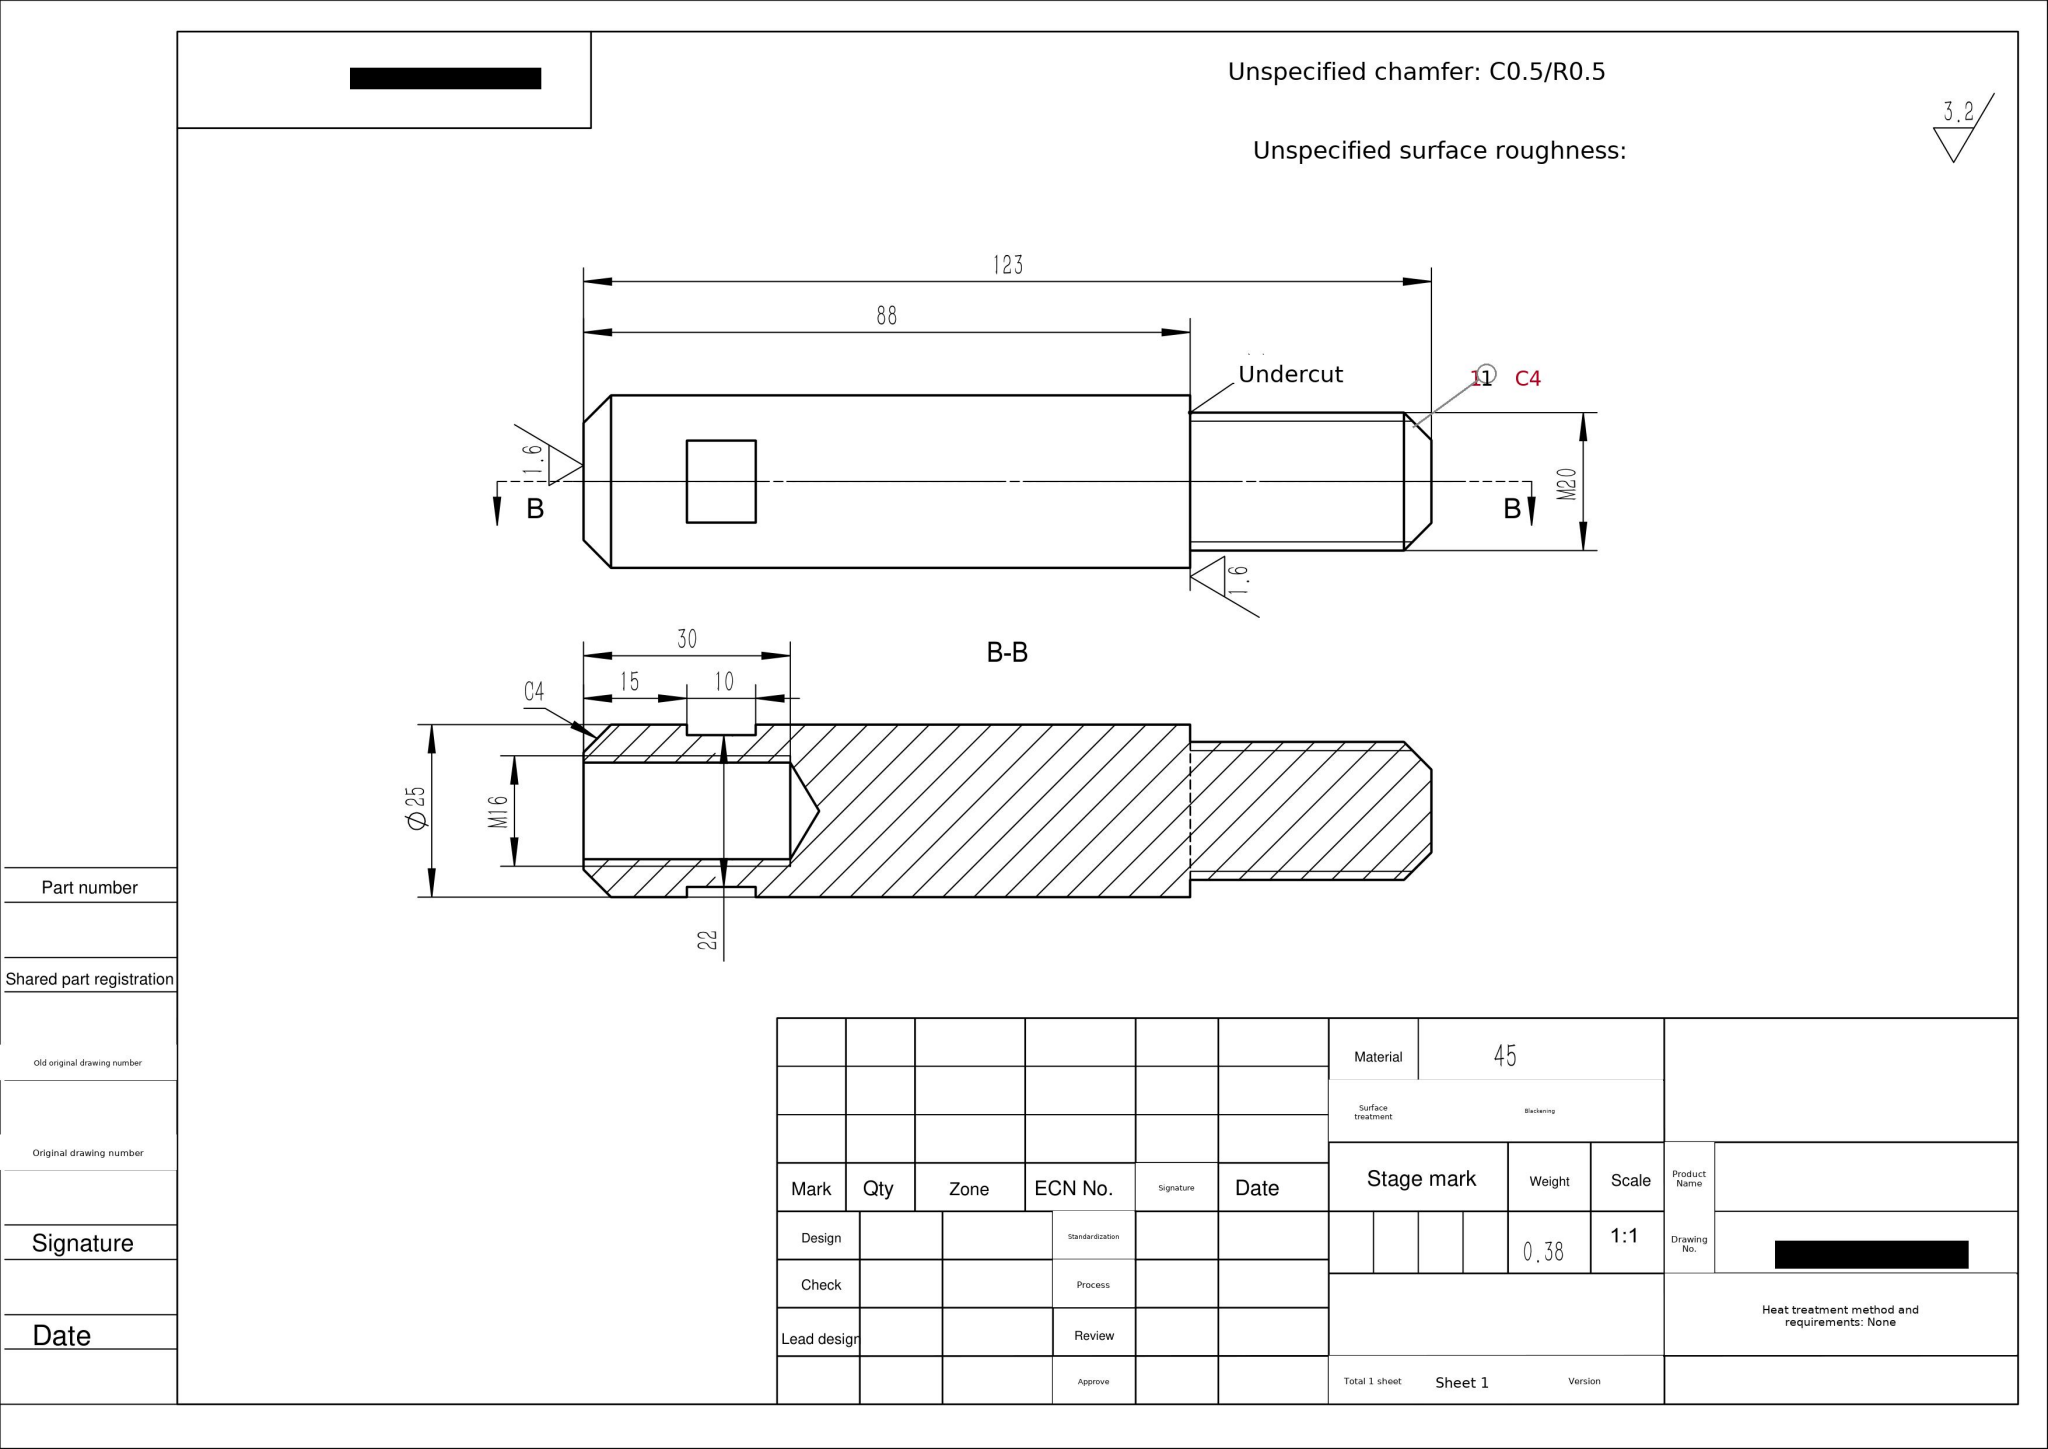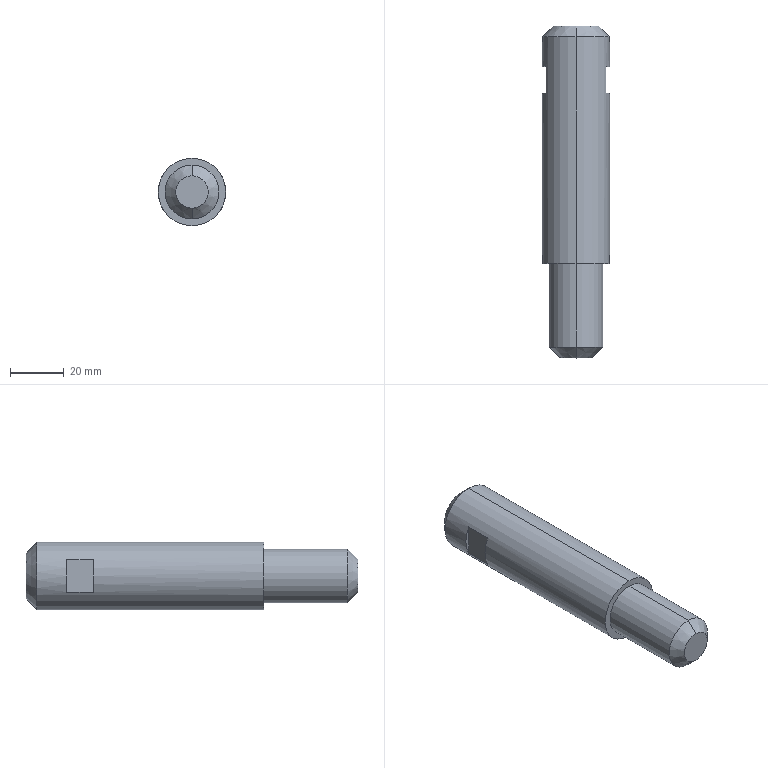Part | SolidWorks | mm | material 45 | 1 solid | 21 faces | box 25 x 123 x 25 mm | volume 48121 mm3 | plane 9 | cylinder 6 | cone 6 | commonest cylinder face diameters 14 x2 20 x2 25 x2
build123d program:
from build123d import *

# Parameters (mm, degrees)
SKETCH1_R              = 12.5
BOSS_EXTRUDE1_DEPTH    = 123
SKETCH2_OUTSIDE_W      = 52.596
SKETCH2_OUTSIDE_H      = 52.596
SKETCH2_OUTSIDE_R      = 10
CUT_EXTRUDE1_DEPTH     = 35
CHAMFER1_SIZE          = 4
M16_TAPPED_HOLE1_D     = 14
M16_TAPPED_HOLE1_DEPTH = 30
M16_TAPPED_HOLE1_TIP   = 4.206
CUT_EXTRUDE2_START     = -15
SKETCH8_OUTSIDE_W      = 52.596
SKETCH8_OUTSIDE_H      = 52.596
SKETCH8_OUTSIDE_W_2    = 22
SKETCH8_OUTSIDE_H_2    = 26.005
CUT_EXTRUDE2_DEPTH     = 10


with BuildPart() as part:
    # Sketch1 → Boss-Extrude1 (new body)
    with BuildSketch(Plane(origin=(0, 0, 0), x_dir=(1, 0, 0), z_dir=(0, 1, 0))):
        with Locations(Location((0, 0, 0), (0, 0, 270))):
            Circle(SKETCH1_R)
    extrude(amount=BOSS_EXTRUDE1_DEPTH)

    # Sketch2 outside → Cut-Extrude1 (cut)
    with BuildSketch(Plane.XZ):
        Rectangle(SKETCH2_OUTSIDE_W, SKETCH2_OUTSIDE_H)
        with Locations(Location((0, 0, 0), (0, 0, 270))):
            Circle(SKETCH2_OUTSIDE_R, mode=Mode.SUBTRACT)
    extrude(amount=-CUT_EXTRUDE1_DEPTH, mode=Mode.SUBTRACT)

    # Chamfer1
    chamfer1_edges = [part.edges().sort_by_distance(p)[0] for p in [
        (0, 0, 10),
        (0, 123, -12.5),
    ]]
    chamfer(chamfer1_edges, length=CHAMFER1_SIZE)

    # M16 Tapped Hole1
    with Locations(Plane(origin=(0, 123, 0), x_dir=(1, 0, 0), z_dir=(0, 1, 0))):
        with Locations((0, 0)):
            Hole(M16_TAPPED_HOLE1_D / 2, depth=M16_TAPPED_HOLE1_DEPTH)
            with Locations((0, 0, -(M16_TAPPED_HOLE1_DEPTH + M16_TAPPED_HOLE1_TIP / 2))):  # 118° drill point
                Cone(0, M16_TAPPED_HOLE1_D / 2, M16_TAPPED_HOLE1_TIP, mode=Mode.SUBTRACT)

    # Sketch8 outside → Cut-Extrude2 (cut)
    with BuildSketch(Plane(origin=(0, 123, 0), x_dir=(1, 0, 0), z_dir=(0, 1, 0)).offset(CUT_EXTRUDE2_START)):
        Rectangle(SKETCH8_OUTSIDE_W, SKETCH8_OUTSIDE_H)
        Rectangle(SKETCH8_OUTSIDE_W_2, SKETCH8_OUTSIDE_H_2, mode=Mode.SUBTRACT)
    extrude(amount=-CUT_EXTRUDE2_DEPTH, mode=Mode.SUBTRACT)


solid = part.part
STEP:
#1=CARTESIAN_POINT('',(0.,93.,-7.));
#2=VERTEX_POINT('',#1);
#3=CARTESIAN_POINT('',(0.,93.,7.));
#4=VERTEX_POINT('',#3);
#5=CARTESIAN_POINT('',(0.,93.,0.));
#6=DIRECTION('',(0.,1.,0.));
#7=DIRECTION('',(0.,0.,1.));
#8=AXIS2_PLACEMENT_3D('',#5,#6,#7);
#9=CIRCLE('',#8,7.);
#10=EDGE_CURVE('',#2,#4,#9,.T.);
#11=ORIENTED_EDGE('',*,*,#10,.F.);
#12=CARTESIAN_POINT('',(0.,123.,-7.));
#13=VERTEX_POINT('',#12);
#14=CARTESIAN_POINT('',(0.,123.,-7.));
#15=DIRECTION('',(0.,1.,0.));
#16=VECTOR('',#15,1000.);
#17=LINE('',#14,#16);
#18=EDGE_CURVE('',#2,#13,#17,.T.);
#19=ORIENTED_EDGE('',*,*,#18,.T.);
#20=CARTESIAN_POINT('',(0.,123.,7.));
#21=VERTEX_POINT('',#20);
#22=CARTESIAN_POINT('',(0.,123.,0.));
#23=DIRECTION('',(0.,1.,0.));
#24=DIRECTION('',(0.,0.,1.));
#25=AXIS2_PLACEMENT_3D('',#22,#23,#24);
#26=CIRCLE('',#25,7.);
#27=EDGE_CURVE('',#13,#21,#26,.T.);
#28=ORIENTED_EDGE('',*,*,#27,.T.);
#29=CARTESIAN_POINT('',(0.,123.,7.));
#30=DIRECTION('',(0.,1.,0.));
#31=VECTOR('',#30,1000.);
#32=LINE('',#29,#31);
#33=EDGE_CURVE('',#4,#21,#32,.T.);
#34=ORIENTED_EDGE('',*,*,#33,.F.);
#35=EDGE_LOOP('',(#11,#19,#28,#34));
#36=FACE_OUTER_BOUND('',#35,.T.);
#37=CARTESIAN_POINT('',(0.,123.,0.));
#38=DIRECTION('',(0.,1.,0.));
#39=DIRECTION('',(0.,0.,1.));
#40=AXIS2_PLACEMENT_3D('',#37,#38,#39);
#41=CYLINDRICAL_SURFACE('',#40,7.);
#42=ADVANCED_FACE('',(#36),#41,.F.);
#43=CARTESIAN_POINT('',(-0.,88.794,0.));
#44=VERTEX_POINT('',#43);
#45=CARTESIAN_POINT('',(0.,93.,7.));
#46=DIRECTION('',(0.,0.515,0.8572));
#47=VECTOR('',#46,1000.);
#48=LINE('',#45,#47);
#49=EDGE_CURVE('',#44,#4,#48,.T.);
#50=ORIENTED_EDGE('',*,*,#49,.F.);
#51=CARTESIAN_POINT('',(0.,93.,-7.));
#52=DIRECTION('',(0.,0.515,-0.8572));
#53=VECTOR('',#52,1000.);
#54=LINE('',#51,#53);
#55=EDGE_CURVE('',#44,#2,#54,.T.);
#56=ORIENTED_EDGE('',*,*,#55,.T.);
#57=ORIENTED_EDGE('',*,*,#10,.T.);
#58=EDGE_LOOP('',(#50,#56,#57));
#59=FACE_OUTER_BOUND('',#58,.T.);
#60=CARTESIAN_POINT('',(0.,93.,0.));
#61=DIRECTION('',(0.,1.,0.));
#62=DIRECTION('',(0.,0.,1.));
#63=AXIS2_PLACEMENT_3D('',#60,#61,#62);
#64=CONICAL_SURFACE('',#63,7.,1.03);
#65=ADVANCED_FACE('',(#59),#64,.F.);
#66=CARTESIAN_POINT('',(0.,0.,-6.));
#67=VERTEX_POINT('',#66);
#68=CARTESIAN_POINT('',(0.,0.,6.));
#69=VERTEX_POINT('',#68);
#70=CARTESIAN_POINT('',(0.,0.,0.));
#71=DIRECTION('',(0.,-1.,0.));
#72=DIRECTION('',(0.,0.,1.));
#73=AXIS2_PLACEMENT_3D('',#70,#71,#72);
#74=CIRCLE('',#73,6.);
#75=EDGE_CURVE('',#67,#69,#74,.T.);
#76=ORIENTED_EDGE('',*,*,#75,.F.);
#77=CARTESIAN_POINT('',(0.,4.,-10.));
#78=VERTEX_POINT('',#77);
#79=CARTESIAN_POINT('',(0.,0.,-6.));
#80=DIRECTION('',(0.,0.7071,-0.7071));
#81=VECTOR('',#80,1000.);
#82=LINE('',#79,#81);
#83=EDGE_CURVE('',#67,#78,#82,.T.);
#84=ORIENTED_EDGE('',*,*,#83,.T.);
#85=CARTESIAN_POINT('',(0.,4.,10.));
#86=VERTEX_POINT('',#85);
#87=CARTESIAN_POINT('',(0.,4.,0.));
#88=DIRECTION('',(0.,1.,0.));
#89=DIRECTION('',(0.,0.,1.));
#90=AXIS2_PLACEMENT_3D('',#87,#88,#89);
#91=CIRCLE('',#90,10.);
#92=EDGE_CURVE('',#86,#78,#91,.T.);
#93=ORIENTED_EDGE('',*,*,#92,.F.);
#94=CARTESIAN_POINT('',(0.,0.,6.));
#95=DIRECTION('',(0.,0.7071,0.7071));
#96=VECTOR('',#95,1000.);
#97=LINE('',#94,#96);
#98=EDGE_CURVE('',#69,#86,#97,.T.);
#99=ORIENTED_EDGE('',*,*,#98,.F.);
#100=EDGE_LOOP('',(#76,#84,#93,#99));
#101=FACE_OUTER_BOUND('',#100,.T.);
#102=CARTESIAN_POINT('',(0.,0.,0.));
#103=DIRECTION('',(0.,1.,0.));
#104=DIRECTION('',(0.,0.,1.));
#105=AXIS2_PLACEMENT_3D('',#102,#103,#104);
#106=CONICAL_SURFACE('',#105,6.,0.7854);
#107=ADVANCED_FACE('',(#101),#106,.T.);
#108=CARTESIAN_POINT('',(0.,123.,8.5));
#109=VERTEX_POINT('',#108);
#110=CARTESIAN_POINT('',(0.,123.,-8.5));
#111=VERTEX_POINT('',#110);
#112=CARTESIAN_POINT('',(0.,123.,0.));
#113=DIRECTION('',(0.,1.,0.));
#114=DIRECTION('',(0.,0.,1.));
#115=AXIS2_PLACEMENT_3D('',#112,#113,#114);
#116=CIRCLE('',#115,8.5);
#117=EDGE_CURVE('',#109,#111,#116,.T.);
#118=ORIENTED_EDGE('',*,*,#117,.F.);
#119=CARTESIAN_POINT('',(0.,119.,12.5));
#120=VERTEX_POINT('',#119);
#121=CARTESIAN_POINT('',(0.,123.,8.5));
#122=DIRECTION('',(0.,-0.7071,0.7071));
#123=VECTOR('',#122,1000.);
#124=LINE('',#121,#123);
#125=EDGE_CURVE('',#109,#120,#124,.T.);
#126=ORIENTED_EDGE('',*,*,#125,.T.);
#127=CARTESIAN_POINT('',(0.,119.,-12.5));
#128=VERTEX_POINT('',#127);
#129=CARTESIAN_POINT('',(0.,119.,0.));
#130=DIRECTION('',(0.,-1.,0.));
#131=DIRECTION('',(0.,0.,1.));
#132=AXIS2_PLACEMENT_3D('',#129,#130,#131);
#133=CIRCLE('',#132,12.5);
#134=EDGE_CURVE('',#128,#120,#133,.T.);
#135=ORIENTED_EDGE('',*,*,#134,.F.);
#136=CARTESIAN_POINT('',(0.,123.,-8.5));
#137=DIRECTION('',(0.,-0.7071,-0.7071));
#138=VECTOR('',#137,1000.);
#139=LINE('',#136,#138);
#140=EDGE_CURVE('',#111,#128,#139,.T.);
#141=ORIENTED_EDGE('',*,*,#140,.F.);
#142=EDGE_LOOP('',(#118,#126,#135,#141));
#143=FACE_OUTER_BOUND('',#142,.T.);
#144=CARTESIAN_POINT('',(0.,123.,0.));
#145=DIRECTION('',(0.,-1.,0.));
#146=DIRECTION('',(0.,0.,-1.));
#147=AXIS2_PLACEMENT_3D('',#144,#145,#146);
#148=CONICAL_SURFACE('',#147,8.5,0.7854);
#149=ADVANCED_FACE('',(#143),#148,.T.);
#150=CARTESIAN_POINT('',(0.,35.,-10.));
#151=VERTEX_POINT('',#150);
#152=CARTESIAN_POINT('',(0.,35.,10.));
#153=VERTEX_POINT('',#152);
#154=CARTESIAN_POINT('',(0.,35.,0.));
#155=DIRECTION('',(0.,-1.,0.));
#156=DIRECTION('',(0.,0.,-1.));
#157=AXIS2_PLACEMENT_3D('',#154,#155,#156);
#158=CIRCLE('',#157,10.);
#159=EDGE_CURVE('',#151,#153,#158,.T.);
#160=ORIENTED_EDGE('',*,*,#159,.T.);
#161=CARTESIAN_POINT('',(0.,35.,10.));
#162=DIRECTION('',(0.,-1.,0.));
#163=VECTOR('',#162,1000.);
#164=LINE('',#161,#163);
#165=EDGE_CURVE('',#153,#86,#164,.T.);
#166=ORIENTED_EDGE('',*,*,#165,.T.);
#167=ORIENTED_EDGE('',*,*,#92,.T.);
#168=CARTESIAN_POINT('',(0.,35.,-10.));
#169=DIRECTION('',(0.,-1.,0.));
#170=VECTOR('',#169,1000.);
#171=LINE('',#168,#170);
#172=EDGE_CURVE('',#151,#78,#171,.T.);
#173=ORIENTED_EDGE('',*,*,#172,.F.);
#174=EDGE_LOOP('',(#160,#166,#167,#173));
#175=FACE_OUTER_BOUND('',#174,.T.);
#176=CARTESIAN_POINT('',(0.,35.,0.));
#177=DIRECTION('',(0.,-1.,0.));
#178=DIRECTION('',(0.,0.,-1.));
#179=AXIS2_PLACEMENT_3D('',#176,#177,#178);
#180=CYLINDRICAL_SURFACE('',#179,10.);
#181=ADVANCED_FACE('',(#175),#180,.T.);
#182=CARTESIAN_POINT('',(11.,108.,5.937));
#183=VERTEX_POINT('',#182);
#184=CARTESIAN_POINT('',(11.,98.,5.937));
#185=VERTEX_POINT('',#184);
#186=CARTESIAN_POINT('',(11.,123.,5.937));
#187=DIRECTION('',(0.,-1.,0.));
#188=VECTOR('',#187,1000.);
#189=LINE('',#186,#188);
#190=EDGE_CURVE('',#183,#185,#189,.T.);
#191=ORIENTED_EDGE('',*,*,#190,.F.);
#192=CARTESIAN_POINT('',(11.,108.,-5.937));
#193=VERTEX_POINT('',#192);
#194=CARTESIAN_POINT('',(0.,108.,0.));
#195=DIRECTION('',(0.,1.,0.));
#196=DIRECTION('',(0.,0.,1.));
#197=AXIS2_PLACEMENT_3D('',#194,#195,#196);
#198=CIRCLE('',#197,12.5);
#199=EDGE_CURVE('',#183,#193,#198,.T.);
#200=ORIENTED_EDGE('',*,*,#199,.T.);
#201=CARTESIAN_POINT('',(11.,98.,-5.937));
#202=VERTEX_POINT('',#201);
#203=CARTESIAN_POINT('',(11.,123.,-5.937));
#204=DIRECTION('',(0.,1.,0.));
#205=VECTOR('',#204,1000.);
#206=LINE('',#203,#205);
#207=EDGE_CURVE('',#202,#193,#206,.T.);
#208=ORIENTED_EDGE('',*,*,#207,.F.);
#209=CARTESIAN_POINT('',(0.,98.,0.));
#210=DIRECTION('',(0.,1.,0.));
#211=DIRECTION('',(0.,0.,1.));
#212=AXIS2_PLACEMENT_3D('',#209,#210,#211);
#213=CIRCLE('',#212,12.5);
#214=EDGE_CURVE('',#185,#202,#213,.T.);
#215=ORIENTED_EDGE('',*,*,#214,.F.);
#216=EDGE_LOOP('',(#191,#200,#208,#215));
#217=FACE_BOUND('',#216,.T.);
#218=ORIENTED_EDGE('',*,*,#134,.T.);
#219=CARTESIAN_POINT('',(0.,35.,12.5));
#220=VERTEX_POINT('',#219);
#221=CARTESIAN_POINT('',(0.,123.,12.5));
#222=DIRECTION('',(0.,-1.,0.));
#223=VECTOR('',#222,1000.);
#224=LINE('',#221,#223);
#225=EDGE_CURVE('',#120,#220,#224,.T.);
#226=ORIENTED_EDGE('',*,*,#225,.T.);
#227=CARTESIAN_POINT('',(0.,35.,-12.5));
#228=VERTEX_POINT('',#227);
#229=CARTESIAN_POINT('',(0.,35.,0.));
#230=DIRECTION('',(0.,-1.,0.));
#231=DIRECTION('',(0.,0.,-1.));
#232=AXIS2_PLACEMENT_3D('',#229,#230,#231);
#233=CIRCLE('',#232,12.5);
#234=EDGE_CURVE('',#228,#220,#233,.T.);
#235=ORIENTED_EDGE('',*,*,#234,.F.);
#236=CARTESIAN_POINT('',(0.,123.,-12.5));
#237=DIRECTION('',(0.,-1.,0.));
#238=VECTOR('',#237,1000.);
#239=LINE('',#236,#238);
#240=EDGE_CURVE('',#128,#228,#239,.T.);
#241=ORIENTED_EDGE('',*,*,#240,.F.);
#242=EDGE_LOOP('',(#218,#226,#235,#241));
#243=FACE_OUTER_BOUND('',#242,.T.);
#244=CARTESIAN_POINT('',(0.,123.,0.));
#245=DIRECTION('',(0.,-1.,0.));
#246=DIRECTION('',(0.,0.,-1.));
#247=AXIS2_PLACEMENT_3D('',#244,#245,#246);
#248=CYLINDRICAL_SURFACE('',#247,12.5);
#249=ADVANCED_FACE('',(#217,#243),#248,.T.);
#250=ORIENTED_EDGE('',*,*,#225,.F.);
#251=CARTESIAN_POINT('',(0.,119.,0.));
#252=DIRECTION('',(0.,-1.,0.));
#253=DIRECTION('',(0.,0.,1.));
#254=AXIS2_PLACEMENT_3D('',#251,#252,#253);
#255=CIRCLE('',#254,12.5);
#256=EDGE_CURVE('',#120,#128,#255,.T.);
#257=ORIENTED_EDGE('',*,*,#256,.T.);
#258=ORIENTED_EDGE('',*,*,#240,.T.);
#259=CARTESIAN_POINT('',(0.,35.,0.));
#260=DIRECTION('',(0.,-1.,0.));
#261=DIRECTION('',(0.,0.,-1.));
#262=AXIS2_PLACEMENT_3D('',#259,#260,#261);
#263=CIRCLE('',#262,12.5);
#264=EDGE_CURVE('',#220,#228,#263,.T.);
#265=ORIENTED_EDGE('',*,*,#264,.F.);
#266=EDGE_LOOP('',(#250,#257,#258,#265));
#267=FACE_OUTER_BOUND('',#266,.T.);
#268=CARTESIAN_POINT('',(-11.,108.,-5.937));
#269=VERTEX_POINT('',#268);
#270=CARTESIAN_POINT('',(-11.,98.,-5.937));
#271=VERTEX_POINT('',#270);
#272=CARTESIAN_POINT('',(-11.,123.,-5.937));
#273=DIRECTION('',(0.,-1.,0.));
#274=VECTOR('',#273,1000.);
#275=LINE('',#272,#274);
#276=EDGE_CURVE('',#269,#271,#275,.T.);
#277=ORIENTED_EDGE('',*,*,#276,.F.);
#278=CARTESIAN_POINT('',(-11.,108.,5.937));
#279=VERTEX_POINT('',#278);
#280=CARTESIAN_POINT('',(0.,108.,0.));
#281=DIRECTION('',(0.,1.,0.));
#282=DIRECTION('',(0.,0.,1.));
#283=AXIS2_PLACEMENT_3D('',#280,#281,#282);
#284=CIRCLE('',#283,12.5);
#285=EDGE_CURVE('',#269,#279,#284,.T.);
#286=ORIENTED_EDGE('',*,*,#285,.T.);
#287=CARTESIAN_POINT('',(-11.,98.,5.937));
#288=VERTEX_POINT('',#287);
#289=CARTESIAN_POINT('',(-11.,123.,5.937));
#290=DIRECTION('',(0.,1.,0.));
#291=VECTOR('',#290,1000.);
#292=LINE('',#289,#291);
#293=EDGE_CURVE('',#288,#279,#292,.T.);
#294=ORIENTED_EDGE('',*,*,#293,.F.);
#295=CARTESIAN_POINT('',(0.,98.,0.));
#296=DIRECTION('',(0.,1.,0.));
#297=DIRECTION('',(0.,0.,1.));
#298=AXIS2_PLACEMENT_3D('',#295,#296,#297);
#299=CIRCLE('',#298,12.5);
#300=EDGE_CURVE('',#271,#288,#299,.T.);
#301=ORIENTED_EDGE('',*,*,#300,.F.);
#302=EDGE_LOOP('',(#277,#286,#294,#301));
#303=FACE_BOUND('',#302,.T.);
#304=CARTESIAN_POINT('',(0.,123.,0.));
#305=DIRECTION('',(0.,-1.,0.));
#306=DIRECTION('',(0.,0.,-1.));
#307=AXIS2_PLACEMENT_3D('',#304,#305,#306);
#308=CYLINDRICAL_SURFACE('',#307,12.5);
#309=ADVANCED_FACE('',(#267,#303),#308,.T.);
#310=CARTESIAN_POINT('',(0.,123.,0.));
#311=DIRECTION('',(0.,1.,0.));
#312=DIRECTION('',(0.,0.,1.));
#313=AXIS2_PLACEMENT_3D('',#310,#311,#312);
#314=CIRCLE('',#313,7.);
#315=EDGE_CURVE('',#21,#13,#314,.T.);
#316=ORIENTED_EDGE('',*,*,#315,.F.);
#317=ORIENTED_EDGE('',*,*,#27,.F.);
#318=EDGE_LOOP('',(#316,#317));
#319=FACE_BOUND('',#318,.T.);
#320=CARTESIAN_POINT('',(0.,123.,0.));
#321=DIRECTION('',(0.,1.,0.));
#322=DIRECTION('',(0.,0.,1.));
#323=AXIS2_PLACEMENT_3D('',#320,#321,#322);
#324=CIRCLE('',#323,8.5);
#325=EDGE_CURVE('',#111,#109,#324,.T.);
#326=ORIENTED_EDGE('',*,*,#325,.T.);
#327=ORIENTED_EDGE('',*,*,#117,.T.);
#328=EDGE_LOOP('',(#326,#327));
#329=FACE_OUTER_BOUND('',#328,.T.);
#330=CARTESIAN_POINT('',(0.,123.,0.));
#331=DIRECTION('',(0.,1.,0.));
#332=DIRECTION('',(0.,0.,1.));
#333=AXIS2_PLACEMENT_3D('',#330,#331,#332);
#334=PLANE('',#333);
#335=ADVANCED_FACE('',(#319,#329),#334,.T.);
#336=ORIENTED_EDGE('',*,*,#159,.F.);
#337=CARTESIAN_POINT('',(0.,35.,0.));
#338=DIRECTION('',(0.,-1.,0.));
#339=DIRECTION('',(0.,0.,-1.));
#340=AXIS2_PLACEMENT_3D('',#337,#338,#339);
#341=CIRCLE('',#340,10.);
#342=EDGE_CURVE('',#153,#151,#341,.T.);
#343=ORIENTED_EDGE('',*,*,#342,.F.);
#344=EDGE_LOOP('',(#336,#343));
#345=FACE_BOUND('',#344,.T.);
#346=ORIENTED_EDGE('',*,*,#234,.T.);
#347=ORIENTED_EDGE('',*,*,#264,.T.);
#348=EDGE_LOOP('',(#346,#347));
#349=FACE_OUTER_BOUND('',#348,.T.);
#350=CARTESIAN_POINT('',(0.,35.,0.));
#351=DIRECTION('',(0.,-1.,0.));
#352=DIRECTION('',(0.,0.,-1.));
#353=AXIS2_PLACEMENT_3D('',#350,#351,#352);
#354=PLANE('',#353);
#355=ADVANCED_FACE('',(#345,#349),#354,.T.);
#356=ORIENTED_EDGE('',*,*,#165,.F.);
#357=ORIENTED_EDGE('',*,*,#342,.T.);
#358=ORIENTED_EDGE('',*,*,#172,.T.);
#359=CARTESIAN_POINT('',(0.,4.,0.));
#360=DIRECTION('',(0.,1.,0.));
#361=DIRECTION('',(0.,0.,1.));
#362=AXIS2_PLACEMENT_3D('',#359,#360,#361);
#363=CIRCLE('',#362,10.);
#364=EDGE_CURVE('',#78,#86,#363,.T.);
#365=ORIENTED_EDGE('',*,*,#364,.T.);
#366=EDGE_LOOP('',(#356,#357,#358,#365));
#367=FACE_OUTER_BOUND('',#366,.T.);
#368=CARTESIAN_POINT('',(0.,35.,0.));
#369=DIRECTION('',(0.,-1.,0.));
#370=DIRECTION('',(0.,0.,-1.));
#371=AXIS2_PLACEMENT_3D('',#368,#369,#370);
#372=CYLINDRICAL_SURFACE('',#371,10.);
#373=ADVANCED_FACE('',(#367),#372,.T.);
#374=CARTESIAN_POINT('',(0.,0.,0.));
#375=DIRECTION('',(0.,-1.,0.));
#376=DIRECTION('',(0.,0.,1.));
#377=AXIS2_PLACEMENT_3D('',#374,#375,#376);
#378=CIRCLE('',#377,6.);
#379=EDGE_CURVE('',#69,#67,#378,.T.);
#380=ORIENTED_EDGE('',*,*,#379,.T.);
#381=ORIENTED_EDGE('',*,*,#75,.T.);
#382=EDGE_LOOP('',(#380,#381));
#383=FACE_OUTER_BOUND('',#382,.T.);
#384=CARTESIAN_POINT('',(0.,0.,0.));
#385=DIRECTION('',(0.,1.,0.));
#386=DIRECTION('',(0.,0.,1.));
#387=AXIS2_PLACEMENT_3D('',#384,#385,#386);
#388=PLANE('',#387);
#389=ADVANCED_FACE('',(#383),#388,.F.);
#390=ORIENTED_EDGE('',*,*,#125,.F.);
#391=ORIENTED_EDGE('',*,*,#325,.F.);
#392=ORIENTED_EDGE('',*,*,#140,.T.);
#393=ORIENTED_EDGE('',*,*,#256,.F.);
#394=EDGE_LOOP('',(#390,#391,#392,#393));
#395=FACE_OUTER_BOUND('',#394,.T.);
#396=CARTESIAN_POINT('',(0.,123.,0.));
#397=DIRECTION('',(0.,-1.,0.));
#398=DIRECTION('',(0.,0.,-1.));
#399=AXIS2_PLACEMENT_3D('',#396,#397,#398);
#400=CONICAL_SURFACE('',#399,8.5,0.7854);
#401=ADVANCED_FACE('',(#395),#400,.T.);
#402=ORIENTED_EDGE('',*,*,#83,.F.);
#403=ORIENTED_EDGE('',*,*,#379,.F.);
#404=ORIENTED_EDGE('',*,*,#98,.T.);
#405=ORIENTED_EDGE('',*,*,#364,.F.);
#406=EDGE_LOOP('',(#402,#403,#404,#405));
#407=FACE_OUTER_BOUND('',#406,.T.);
#408=CARTESIAN_POINT('',(0.,0.,0.));
#409=DIRECTION('',(0.,1.,0.));
#410=DIRECTION('',(0.,0.,1.));
#411=AXIS2_PLACEMENT_3D('',#408,#409,#410);
#412=CONICAL_SURFACE('',#411,6.,0.7854);
#413=ADVANCED_FACE('',(#407),#412,.T.);
#414=ORIENTED_EDGE('',*,*,#55,.F.);
#415=ORIENTED_EDGE('',*,*,#49,.T.);
#416=CARTESIAN_POINT('',(0.,93.,0.));
#417=DIRECTION('',(0.,1.,0.));
#418=DIRECTION('',(0.,0.,1.));
#419=AXIS2_PLACEMENT_3D('',#416,#417,#418);
#420=CIRCLE('',#419,7.);
#421=EDGE_CURVE('',#4,#2,#420,.T.);
#422=ORIENTED_EDGE('',*,*,#421,.T.);
#423=EDGE_LOOP('',(#414,#415,#422));
#424=FACE_OUTER_BOUND('',#423,.T.);
#425=CARTESIAN_POINT('',(0.,93.,0.));
#426=DIRECTION('',(0.,1.,0.));
#427=DIRECTION('',(0.,0.,1.));
#428=AXIS2_PLACEMENT_3D('',#425,#426,#427);
#429=CONICAL_SURFACE('',#428,7.,1.03);
#430=ADVANCED_FACE('',(#424),#429,.F.);
#431=ORIENTED_EDGE('',*,*,#18,.F.);
#432=ORIENTED_EDGE('',*,*,#421,.F.);
#433=ORIENTED_EDGE('',*,*,#33,.T.);
#434=ORIENTED_EDGE('',*,*,#315,.T.);
#435=EDGE_LOOP('',(#431,#432,#433,#434));
#436=FACE_OUTER_BOUND('',#435,.T.);
#437=CARTESIAN_POINT('',(0.,123.,0.));
#438=DIRECTION('',(0.,1.,0.));
#439=DIRECTION('',(0.,0.,1.));
#440=AXIS2_PLACEMENT_3D('',#437,#438,#439);
#441=CYLINDRICAL_SURFACE('',#440,7.);
#442=ADVANCED_FACE('',(#436),#441,.F.);
#443=ORIENTED_EDGE('',*,*,#190,.T.);
#444=CARTESIAN_POINT('',(11.,98.,-13.002));
#445=DIRECTION('',(-0.,0.,-1.));
#446=VECTOR('',#445,1000.);
#447=LINE('',#444,#446);
#448=EDGE_CURVE('',#185,#202,#447,.T.);
#449=ORIENTED_EDGE('',*,*,#448,.T.);
#450=ORIENTED_EDGE('',*,*,#207,.T.);
#451=CARTESIAN_POINT('',(11.,108.,-13.002));
#452=DIRECTION('',(-0.,0.,-1.));
#453=VECTOR('',#452,1000.);
#454=LINE('',#451,#453);
#455=EDGE_CURVE('',#183,#193,#454,.T.);
#456=ORIENTED_EDGE('',*,*,#455,.F.);
#457=EDGE_LOOP('',(#443,#449,#450,#456));
#458=FACE_OUTER_BOUND('',#457,.T.);
#459=CARTESIAN_POINT('',(11.,98.,-13.002));
#460=DIRECTION('',(1.,0.,-0.));
#461=DIRECTION('',(-0.,0.,-1.));
#462=AXIS2_PLACEMENT_3D('',#459,#460,#461);
#463=PLANE('',#462);
#464=ADVANCED_FACE('',(#458),#463,.T.);
#465=ORIENTED_EDGE('',*,*,#455,.T.);
#466=ORIENTED_EDGE('',*,*,#199,.F.);
#467=EDGE_LOOP('',(#465,#466));
#468=FACE_OUTER_BOUND('',#467,.T.);
#469=CARTESIAN_POINT('',(0.,108.,-0.));
#470=DIRECTION('',(0.,1.,0.));
#471=DIRECTION('',(0.,0.,1.));
#472=AXIS2_PLACEMENT_3D('',#469,#470,#471);
#473=PLANE('',#472);
#474=ADVANCED_FACE('',(#468),#473,.F.);
#475=ORIENTED_EDGE('',*,*,#214,.T.);
#476=ORIENTED_EDGE('',*,*,#448,.F.);
#477=EDGE_LOOP('',(#475,#476));
#478=FACE_OUTER_BOUND('',#477,.T.);
#479=CARTESIAN_POINT('',(0.,98.,-0.));
#480=DIRECTION('',(0.,1.,0.));
#481=DIRECTION('',(0.,0.,1.));
#482=AXIS2_PLACEMENT_3D('',#479,#480,#481);
#483=PLANE('',#482);
#484=ADVANCED_FACE('',(#478),#483,.T.);
#485=ORIENTED_EDGE('',*,*,#300,.T.);
#486=CARTESIAN_POINT('',(-11.,98.,-13.002));
#487=DIRECTION('',(0.,0.,1.));
#488=VECTOR('',#487,1000.);
#489=LINE('',#486,#488);
#490=EDGE_CURVE('',#271,#288,#489,.T.);
#491=ORIENTED_EDGE('',*,*,#490,.F.);
#492=EDGE_LOOP('',(#485,#491));
#493=FACE_OUTER_BOUND('',#492,.T.);
#494=CARTESIAN_POINT('',(0.,98.,-0.));
#495=DIRECTION('',(0.,1.,0.));
#496=DIRECTION('',(0.,0.,1.));
#497=AXIS2_PLACEMENT_3D('',#494,#495,#496);
#498=PLANE('',#497);
#499=ADVANCED_FACE('',(#493),#498,.T.);
#500=CARTESIAN_POINT('',(-11.,108.,-13.002));
#501=DIRECTION('',(0.,0.,1.));
#502=VECTOR('',#501,1000.);
#503=LINE('',#500,#502);
#504=EDGE_CURVE('',#269,#279,#503,.T.);
#505=ORIENTED_EDGE('',*,*,#504,.T.);
#506=ORIENTED_EDGE('',*,*,#285,.F.);
#507=EDGE_LOOP('',(#505,#506));
#508=FACE_OUTER_BOUND('',#507,.T.);
#509=CARTESIAN_POINT('',(0.,108.,-0.));
#510=DIRECTION('',(0.,1.,0.));
#511=DIRECTION('',(0.,0.,1.));
#512=AXIS2_PLACEMENT_3D('',#509,#510,#511);
#513=PLANE('',#512);
#514=ADVANCED_FACE('',(#508),#513,.F.);
#515=ORIENTED_EDGE('',*,*,#276,.T.);
#516=ORIENTED_EDGE('',*,*,#490,.T.);
#517=ORIENTED_EDGE('',*,*,#293,.T.);
#518=ORIENTED_EDGE('',*,*,#504,.F.);
#519=EDGE_LOOP('',(#515,#516,#517,#518));
#520=FACE_OUTER_BOUND('',#519,.T.);
#521=CARTESIAN_POINT('',(-11.,98.,-13.002));
#522=DIRECTION('',(-1.,0.,0.));
#523=DIRECTION('',(0.,0.,1.));
#524=AXIS2_PLACEMENT_3D('',#521,#522,#523);
#525=PLANE('',#524);
#526=ADVANCED_FACE('',(#520),#525,.T.);
#527=CLOSED_SHELL('',(#42,#65,#107,#149,#181,#249,#309,#335,#355,#373,#389,#401,#413,#430,#442,#464,#474,#484,#499,#514,#526));
#528=MANIFOLD_SOLID_BREP('',#527);
#529=CARTESIAN_POINT('',(0.,0.,0.));
#530=DIRECTION('',(0.,0.,1.));
#531=DIRECTION('',(1.,0.,0.));
#532=AXIS2_PLACEMENT_3D('',#529,#530,#531);
#533=(LENGTH_UNIT()NAMED_UNIT(*)SI_UNIT(.MILLI.,.METRE.));
#534=UNCERTAINTY_MEASURE_WITH_UNIT(LENGTH_MEASURE(0.00001),#533,'','');
#535=(NAMED_UNIT(*)PLANE_ANGLE_UNIT()SI_UNIT($,.RADIAN.));
#536=(NAMED_UNIT(*)SI_UNIT($,.STERADIAN.)SOLID_ANGLE_UNIT());
#537=(GEOMETRIC_REPRESENTATION_CONTEXT(3)GLOBAL_UNCERTAINTY_ASSIGNED_CONTEXT((#534))GLOBAL_UNIT_ASSIGNED_CONTEXT((#533,#535,#536))REPRESENTATION_CONTEXT('',''));
#538=ADVANCED_BREP_SHAPE_REPRESENTATION('',(#528,#532),#537);